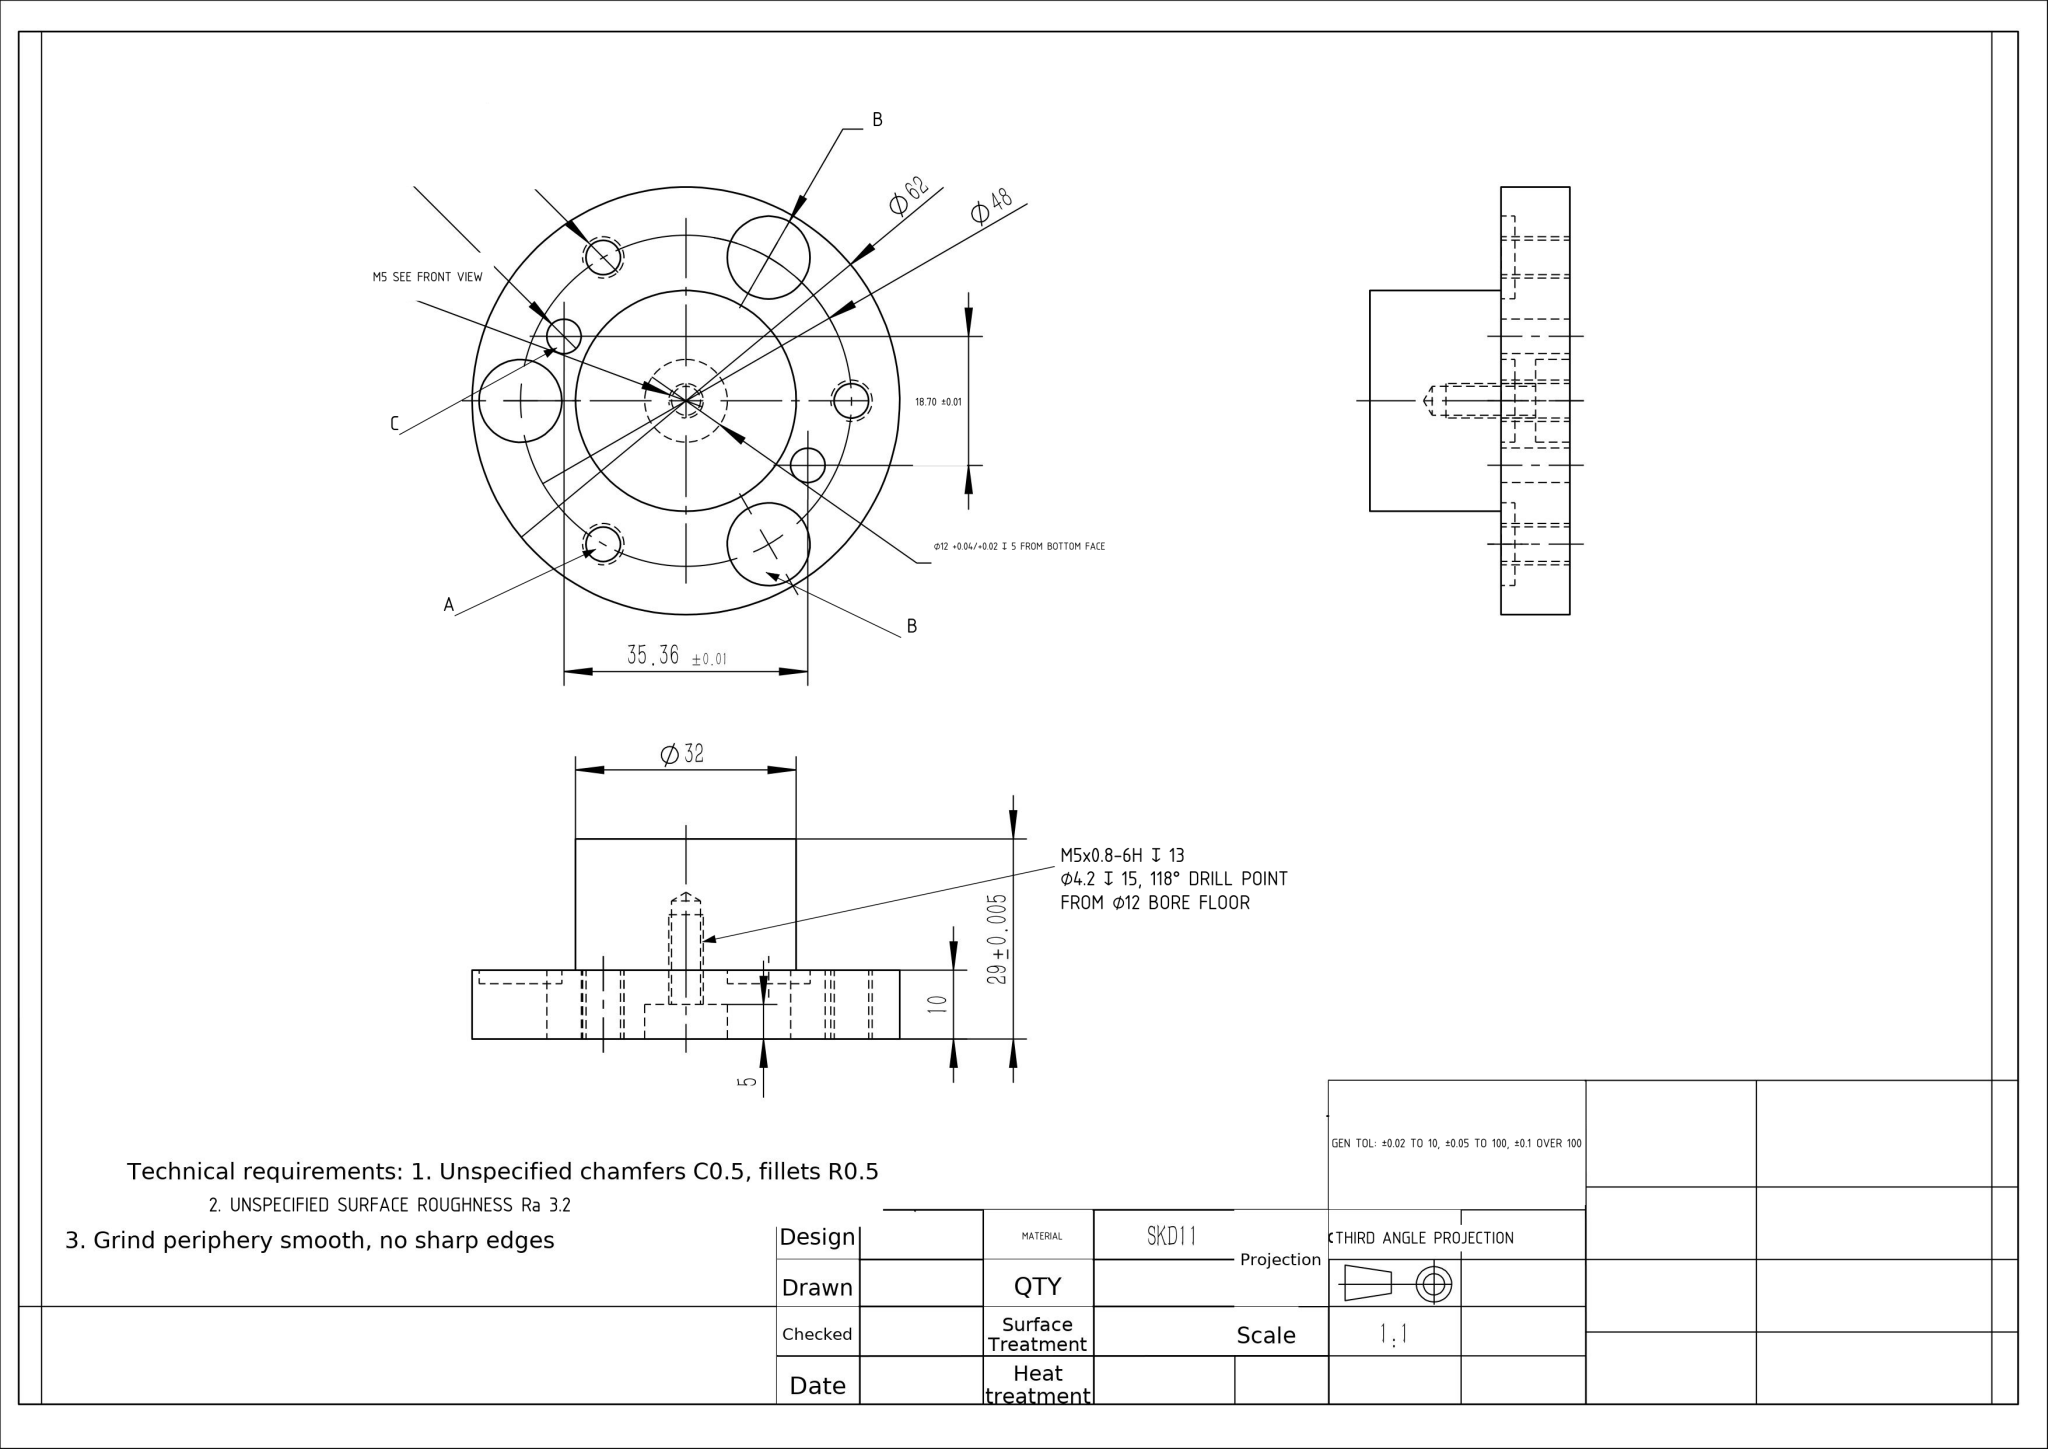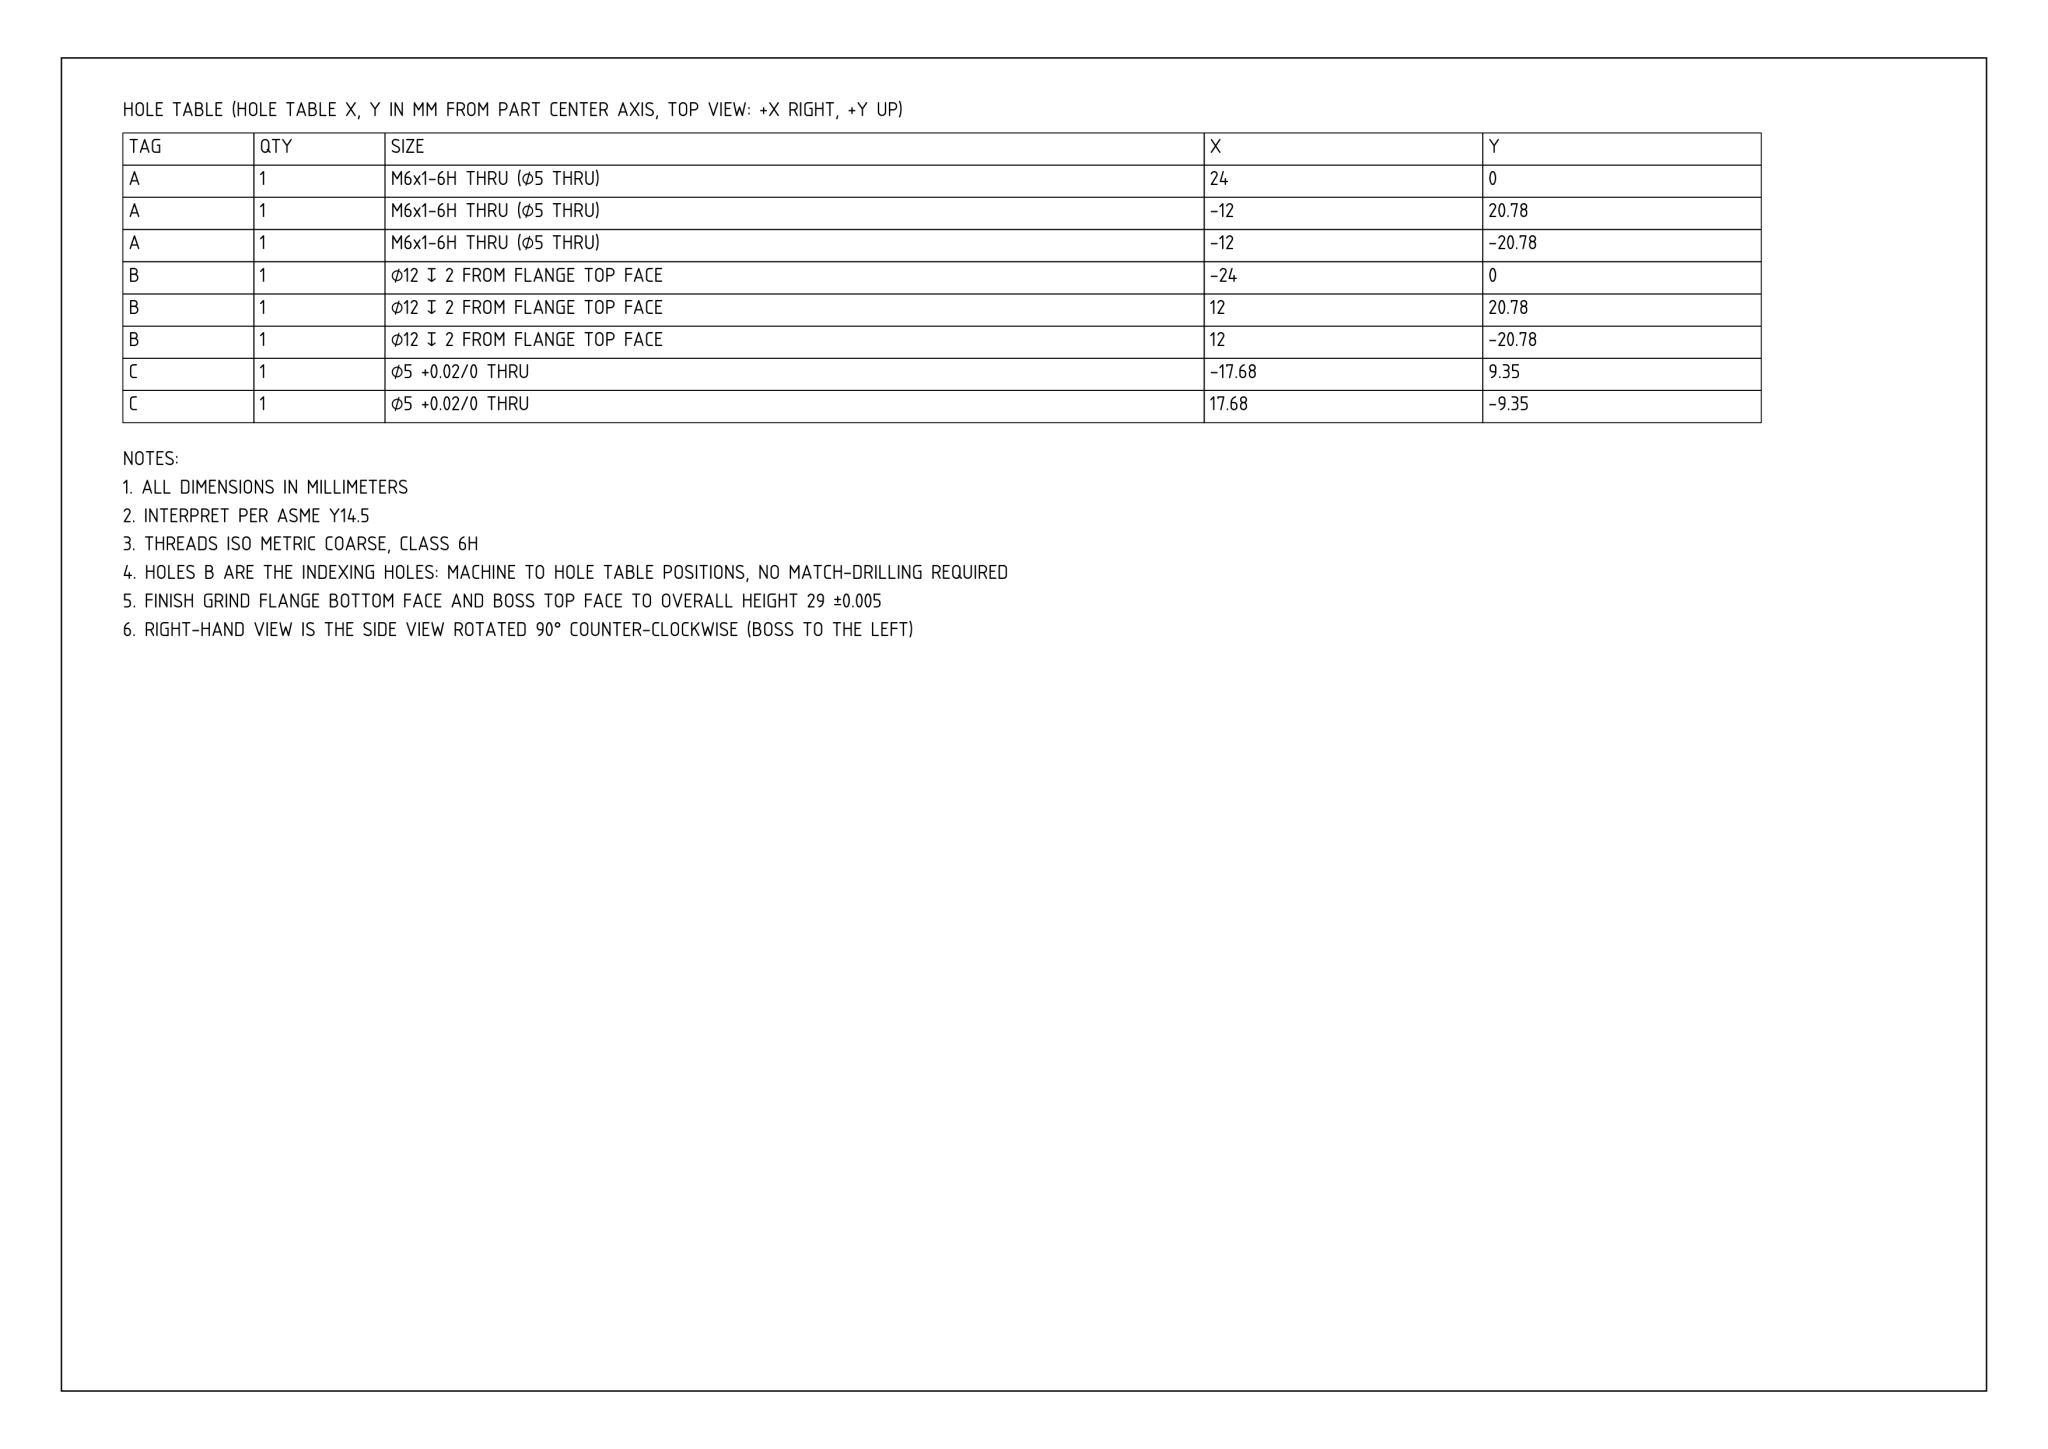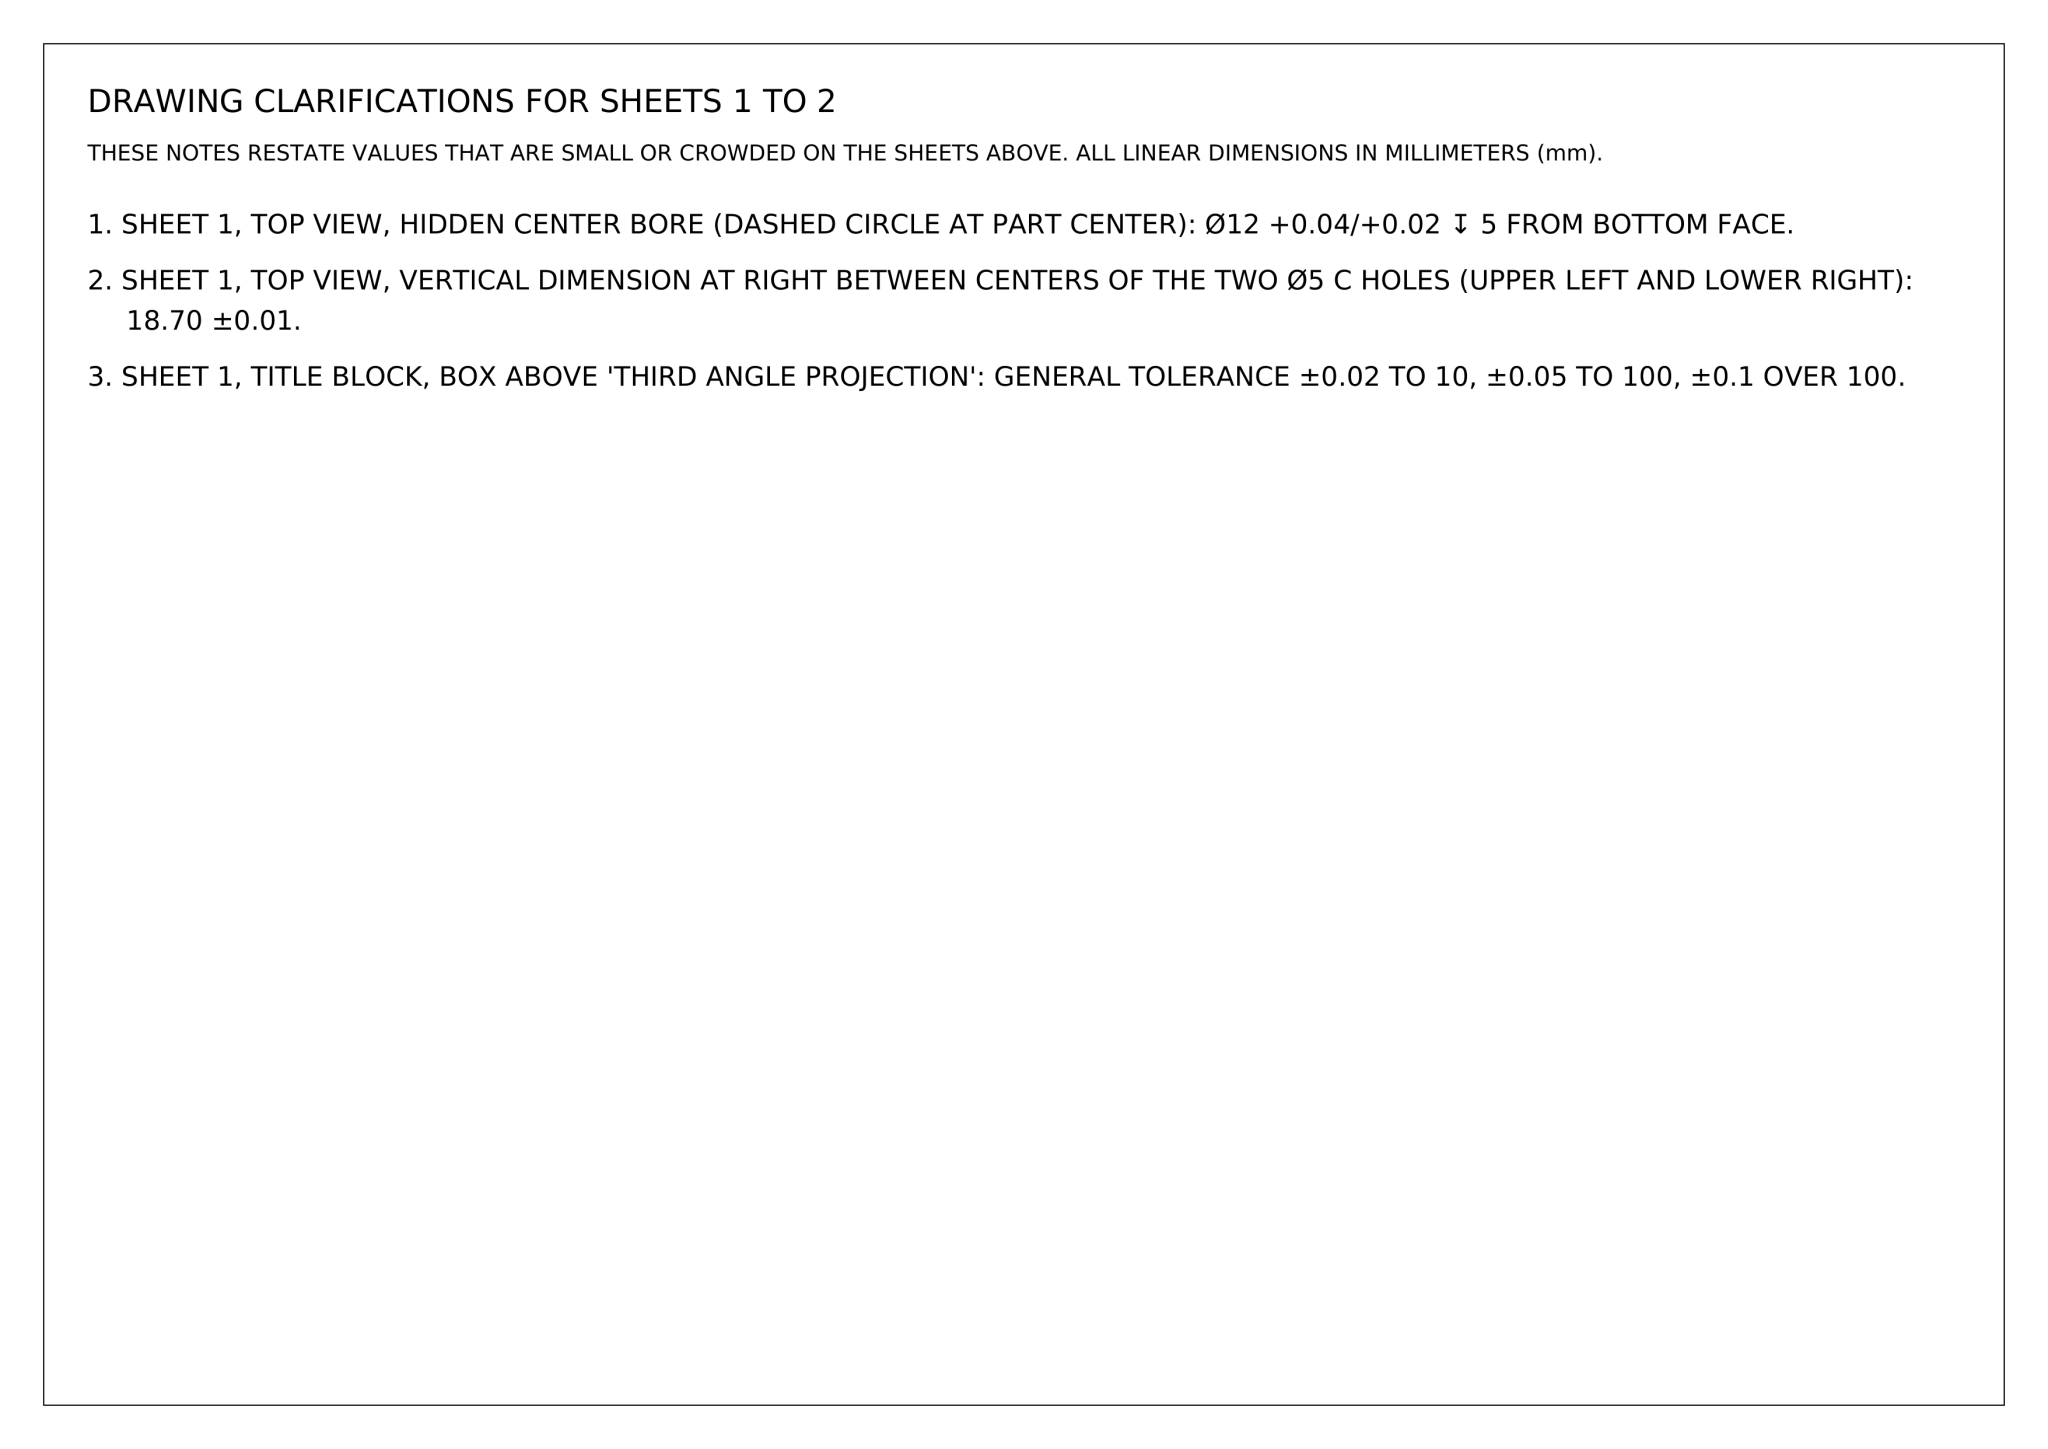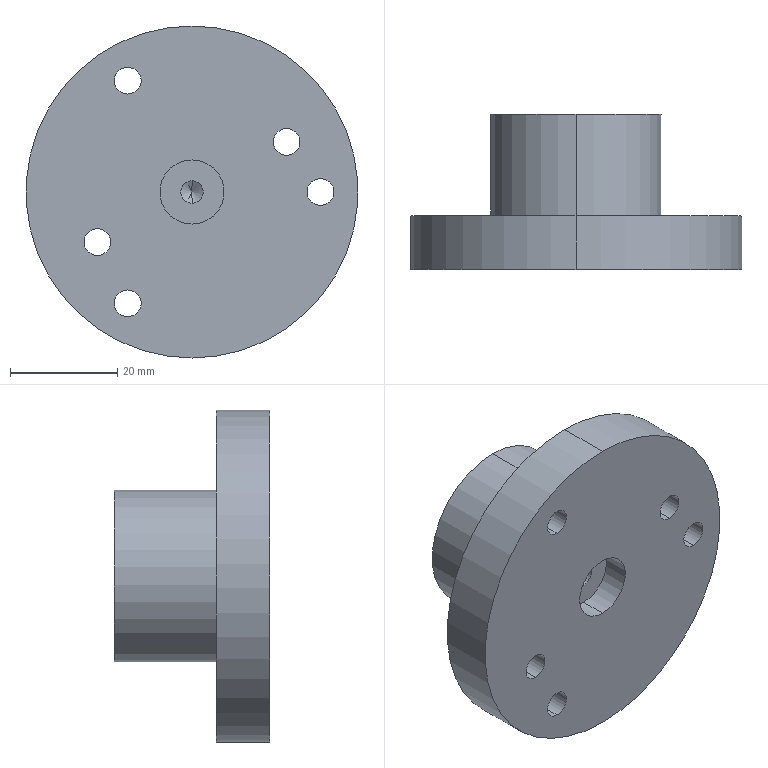Part | NX | mm | 1 solid | 33 faces | box 62 x 29 x 62 mm | volume 43032 mm3 | cylinder 24 | plane 7 | cone 2 | commonest cylinder face diameters 5 x10 12 x8 4.2 x2 32 x2 62 x2